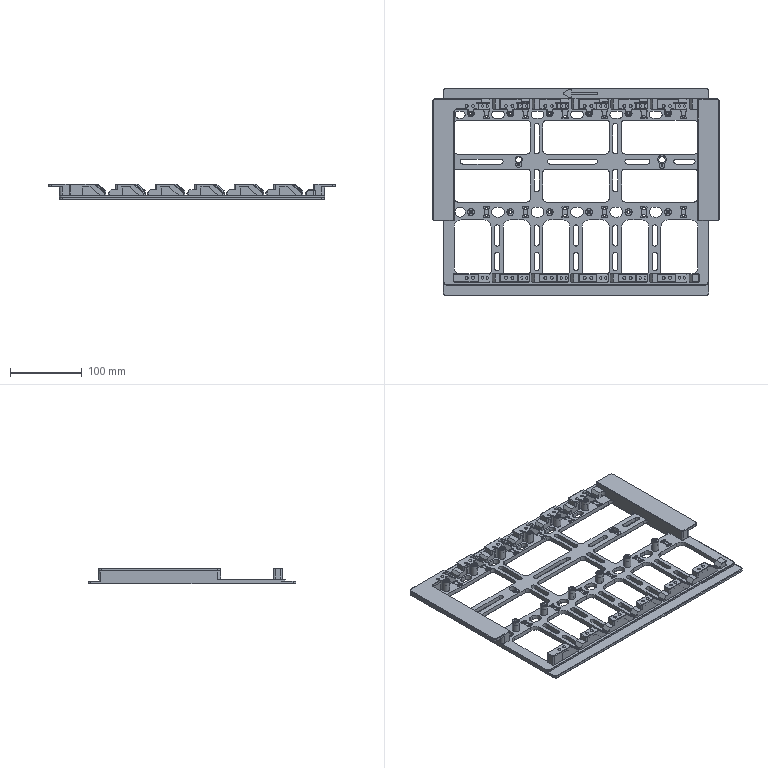CAM job | Mastercam | mm | 94 operations | part box 400 x 290 x 22
1. Facing | 1 - 80 面铣
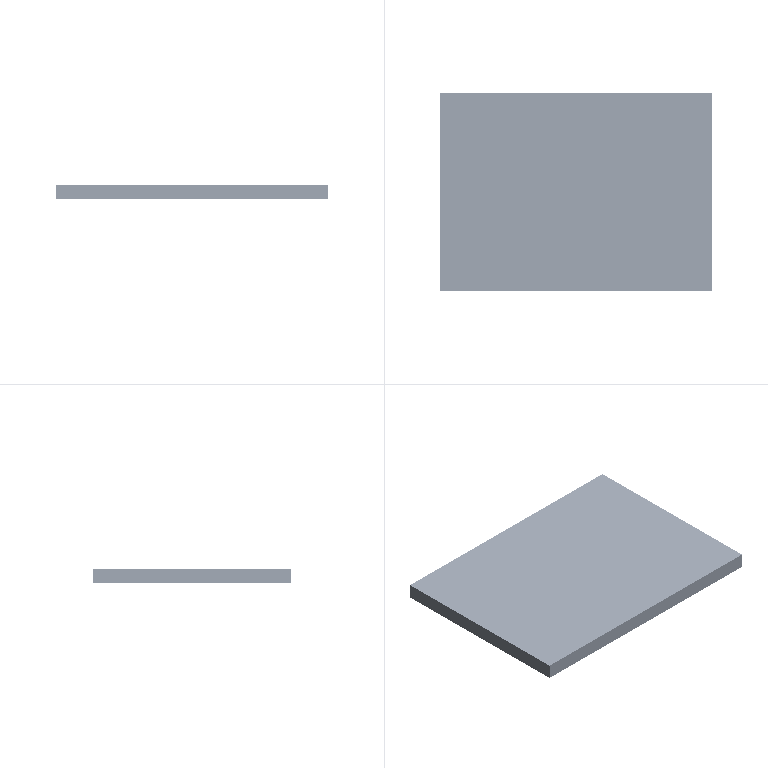2. Surface Rough Pocket | 9 - 10C 平底刀
3. Helix Bore | 6 - 6 平底刀
4. Helix Bore | 6 - 6 平底刀
5. Surface Restmill | 6 - 6 平底刀
6. Contour (2D) | 9 - 10C 平底刀
7. Drill/Counterbore | 2 - 4定位倒角
8. Peck Drill | 18 - 6.8 钻头
9. Drill/Counterbore | 2 - 4定位倒角
10. Peck Drill | 18 - 6.8 钻头
11. Facing | 1 - 80 面铣
12. Contour (2D) | 9 - 10C 平底刀
13. Contour (2D) | 9 - 10C 平底刀
14. Contour (Ramp) | 6 - 6 平底刀
15. Contour (Ramp) | 6 - 6 平底刀
16. Drill/Counterbore | 2 - 4定位倒角
17. Peck Drill | 12 - 2.5 钻头
18. Peck Drill | 19 - 3.5 钻头
19. Surface Rough Pocket | 6 - 6 平底刀
20. 3D High Speed (Waterline) | 8 - 4-R0.5 圆鼻铣刀
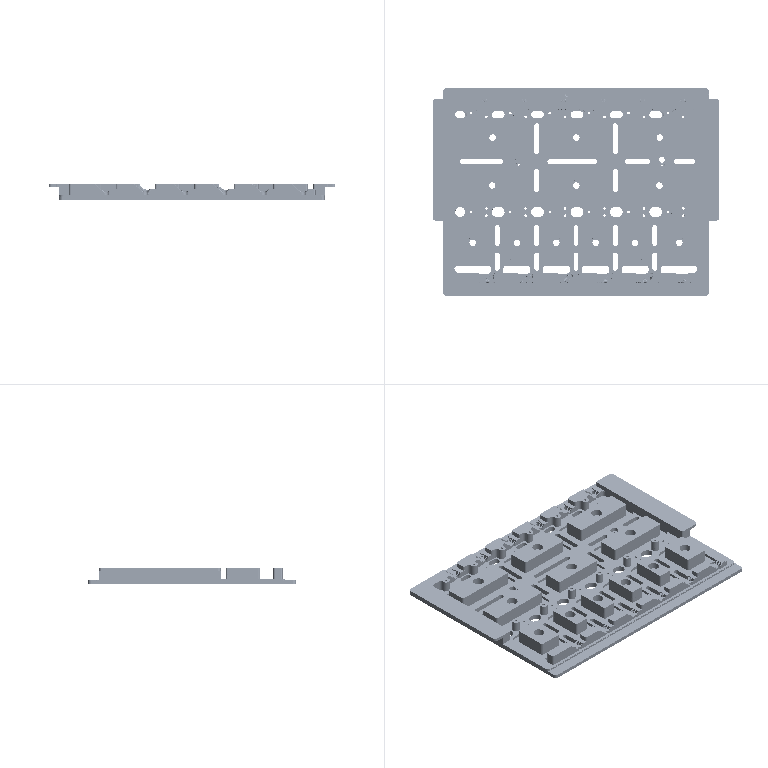21. 3D High Speed (Waterline) | 8 - 4-R0.5 圆鼻铣刀
22. 3D High Speed (Horizontal) | 8 - 4-R0.5 圆鼻铣刀
23. Helix Bore | 7 - 4 平底刀
24. Helix Bore | 7 - 4 平底刀
25. Helix Bore | 20 - 3 平铣刀
26. Helix Bore | 20 - 3 平铣刀
27. Facing | 1 - 80 面铣
28. Contour (2D) | 10 - 10J 平底刀
29. Contour (2D) | 10 - 10J 平底刀
30. Contour (2D) | 6 - 6 平底刀
31. Contour (2D) | 6 - 6 平底刀
32. Model Chamfer | 2 - 4定位倒角
33. Contour (2D chamfer) | 2 - 4定位倒角
34. Contour (2D chamfer) | 2 - 4定位倒角
35. Facing | 9 - 10C 平底刀
36. Contour (2D) | 9 - 10C 平底刀
37. 3D High Speed (Waterline) | 6 - 6 平底刀
38. Contour (Ramp) | 6 - 6 平底刀
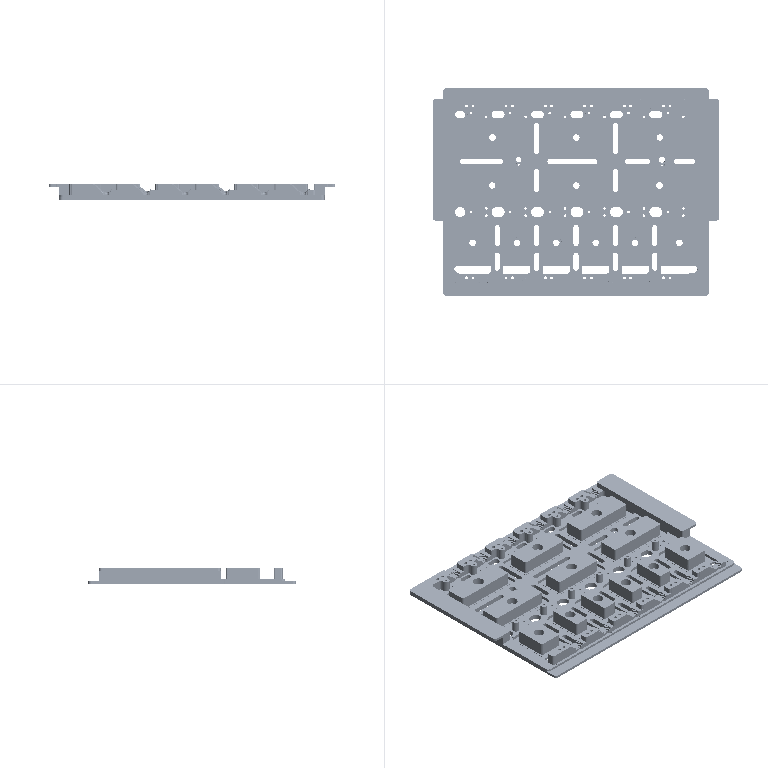39. 3D High Speed (Horizontal) | 6 - 6 平底刀
40. Contour (Remachining) | 20 - 3 平铣刀
41. Helix Bore | 7 - 4 平底刀
42. Pocket (Standard) | 20 - 3 平铣刀
43. Contour (Remachining) | 20 - 3 平铣刀
44. Pocket (Standard) | 20 - 3 平铣刀
45. Contour (Ramp) | 7 - 4 平底刀
46. Contour (Ramp) | 20 - 3 平铣刀
47. Contour (Remachining) | 4 - 2 平铣刀
48. Contour (2D) | 7 - 4 平底刀
49. Contour (Ramp) | 20 - 3 平铣刀
50. Contour (2D) | 20 - 3 平铣刀
51. 3D High Speed (Waterline) | 20 - 3 平铣刀
52. 3D High Speed (Raster) | 5 - 2.0-R0.5 圆鼻铣刀
53. 3D High Speed (Waterline) | 8 - 4-R0.5 圆鼻铣刀
54. 3D High Speed (Waterline rest passes) | 4 - 2 平铣刀
55. Facing | 10 - 10J 平底刀
56. 3D High Speed (Horizontal) | 6 - 6 平底刀
57. Contour (2D) | 6 - 6 平底刀
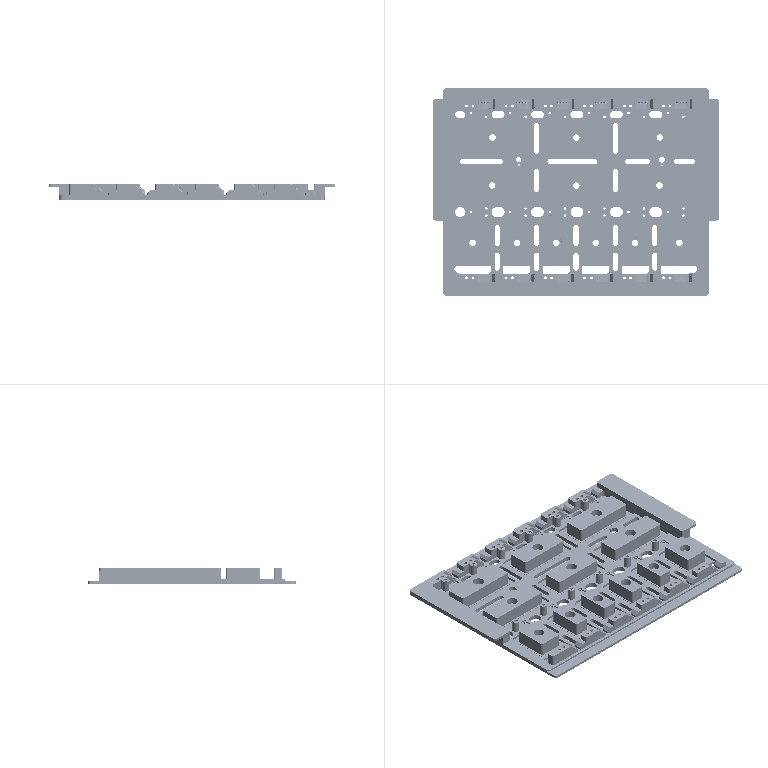58. Contour (2D) | 6 - 6 平底刀
59. Contour (2D) | 6 - 6 平底刀
60. Contour (2D) | 6 - 6 平底刀
61. Contour (2D) | 10 - 10J 平底刀
62. Circle Mill | 7 - 4 平底刀
63. Contour (2D) | 20 - 3 平铣刀
64. Contour (2D) | 7 - 4 平底刀
65. Contour (2D) | 20 - 3 平铣刀
66. Model Chamfer | 2 - 4定位倒角
67. Model Chamfer | 2 - 4定位倒角
68. Model Chamfer | 2 - 4定位倒角
69. Model Chamfer | 2 - 4定位倒角
70. Model Chamfer | 2 - 4定位倒角
71. Chamfer Drill | 2 - 4定位倒角
72. Chamfer Drill | 2 - 4定位倒角
73. Model Chamfer | 2 - 4定位倒角
74. Helix Bore | 20 - 3 平铣刀
75. Helix Bore | 20 - 3 平铣刀
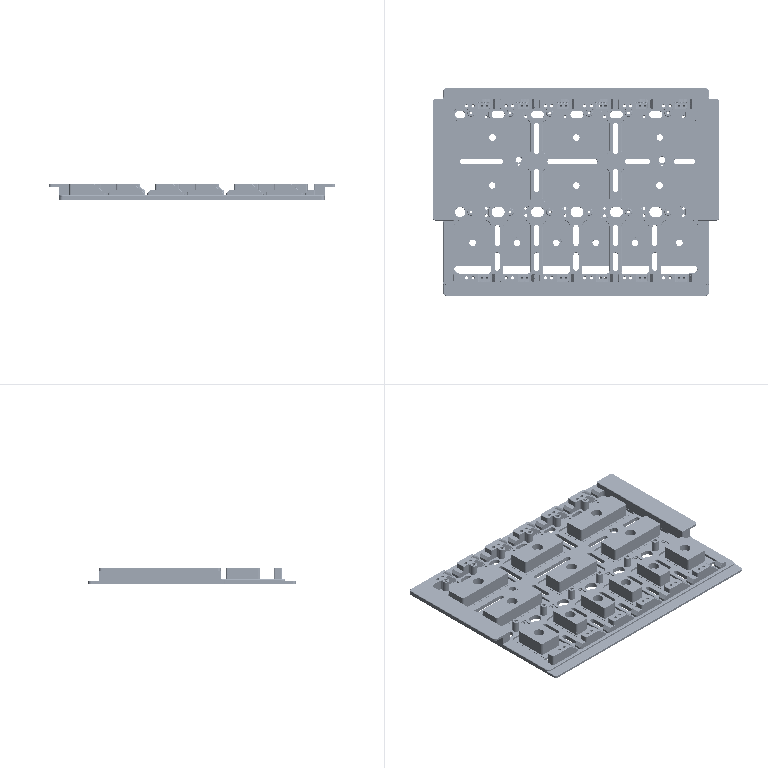76. Contour (Ramp) | 5 - 8 J平底刀
77. Contour (2D) | 6 - 6 平底刀
78. Surface Rough Pocket | 1 - 50 圆鼻铣刀
79. Surface Finish Parallel | 24 - 8 球刀/圆鼻铣刀
80. Drill/Counterbore | 2 - 6定位倒角
81. Peck Drill | 18 - 6.8 钻头
82. Contour (2D chamfer) | 2 - 6定位倒角
83. Tap | 20 - M8 x 1.25 右牙
84. Surface Rough Pocket | 21 - 6 平铣刀
85. 3D High Speed (Waterline) | 21 - 6 平铣刀
86. Helix Bore | 22 - 3 平铣刀
87. Helix Bore | 22 - 3 平铣刀
88. Helix Bore | 22 - 3 平铣刀
89. Helix Bore | 22 - 3 平铣刀
90. Circle Mill | 7 - 4 平底刀
91. Pocket (Standard) | 20 - 3 平铣刀
92. Contour (2D) | 20 - 3 平铣刀
93. Contour (2D) | 7 - 4 平底刀
94. Contour (2D) | 20 - 3 平铣刀